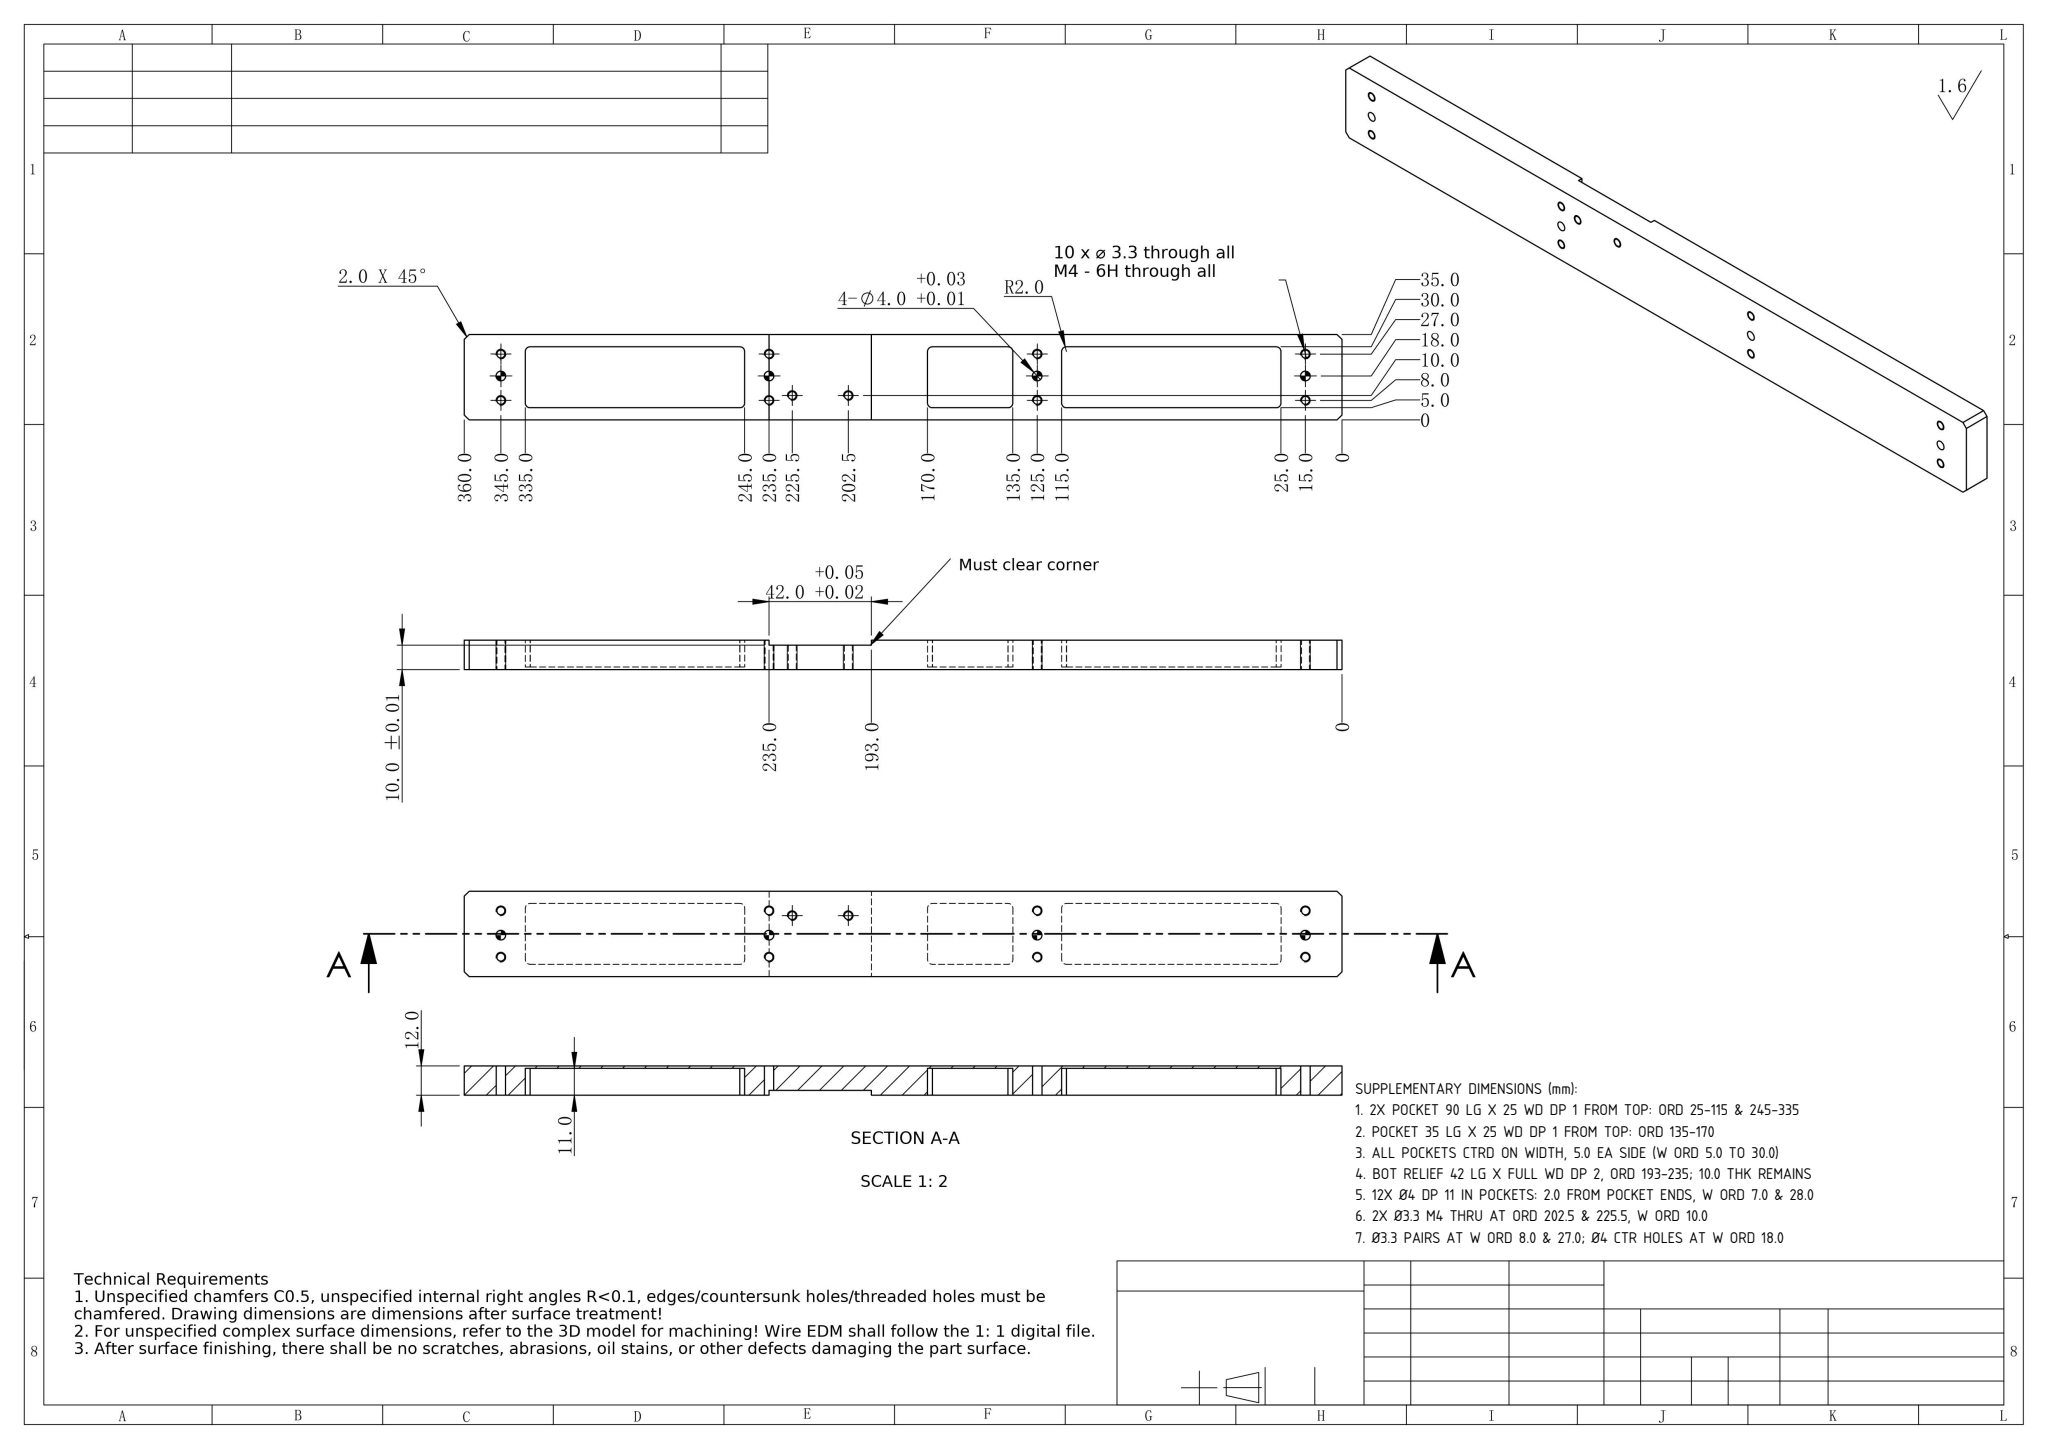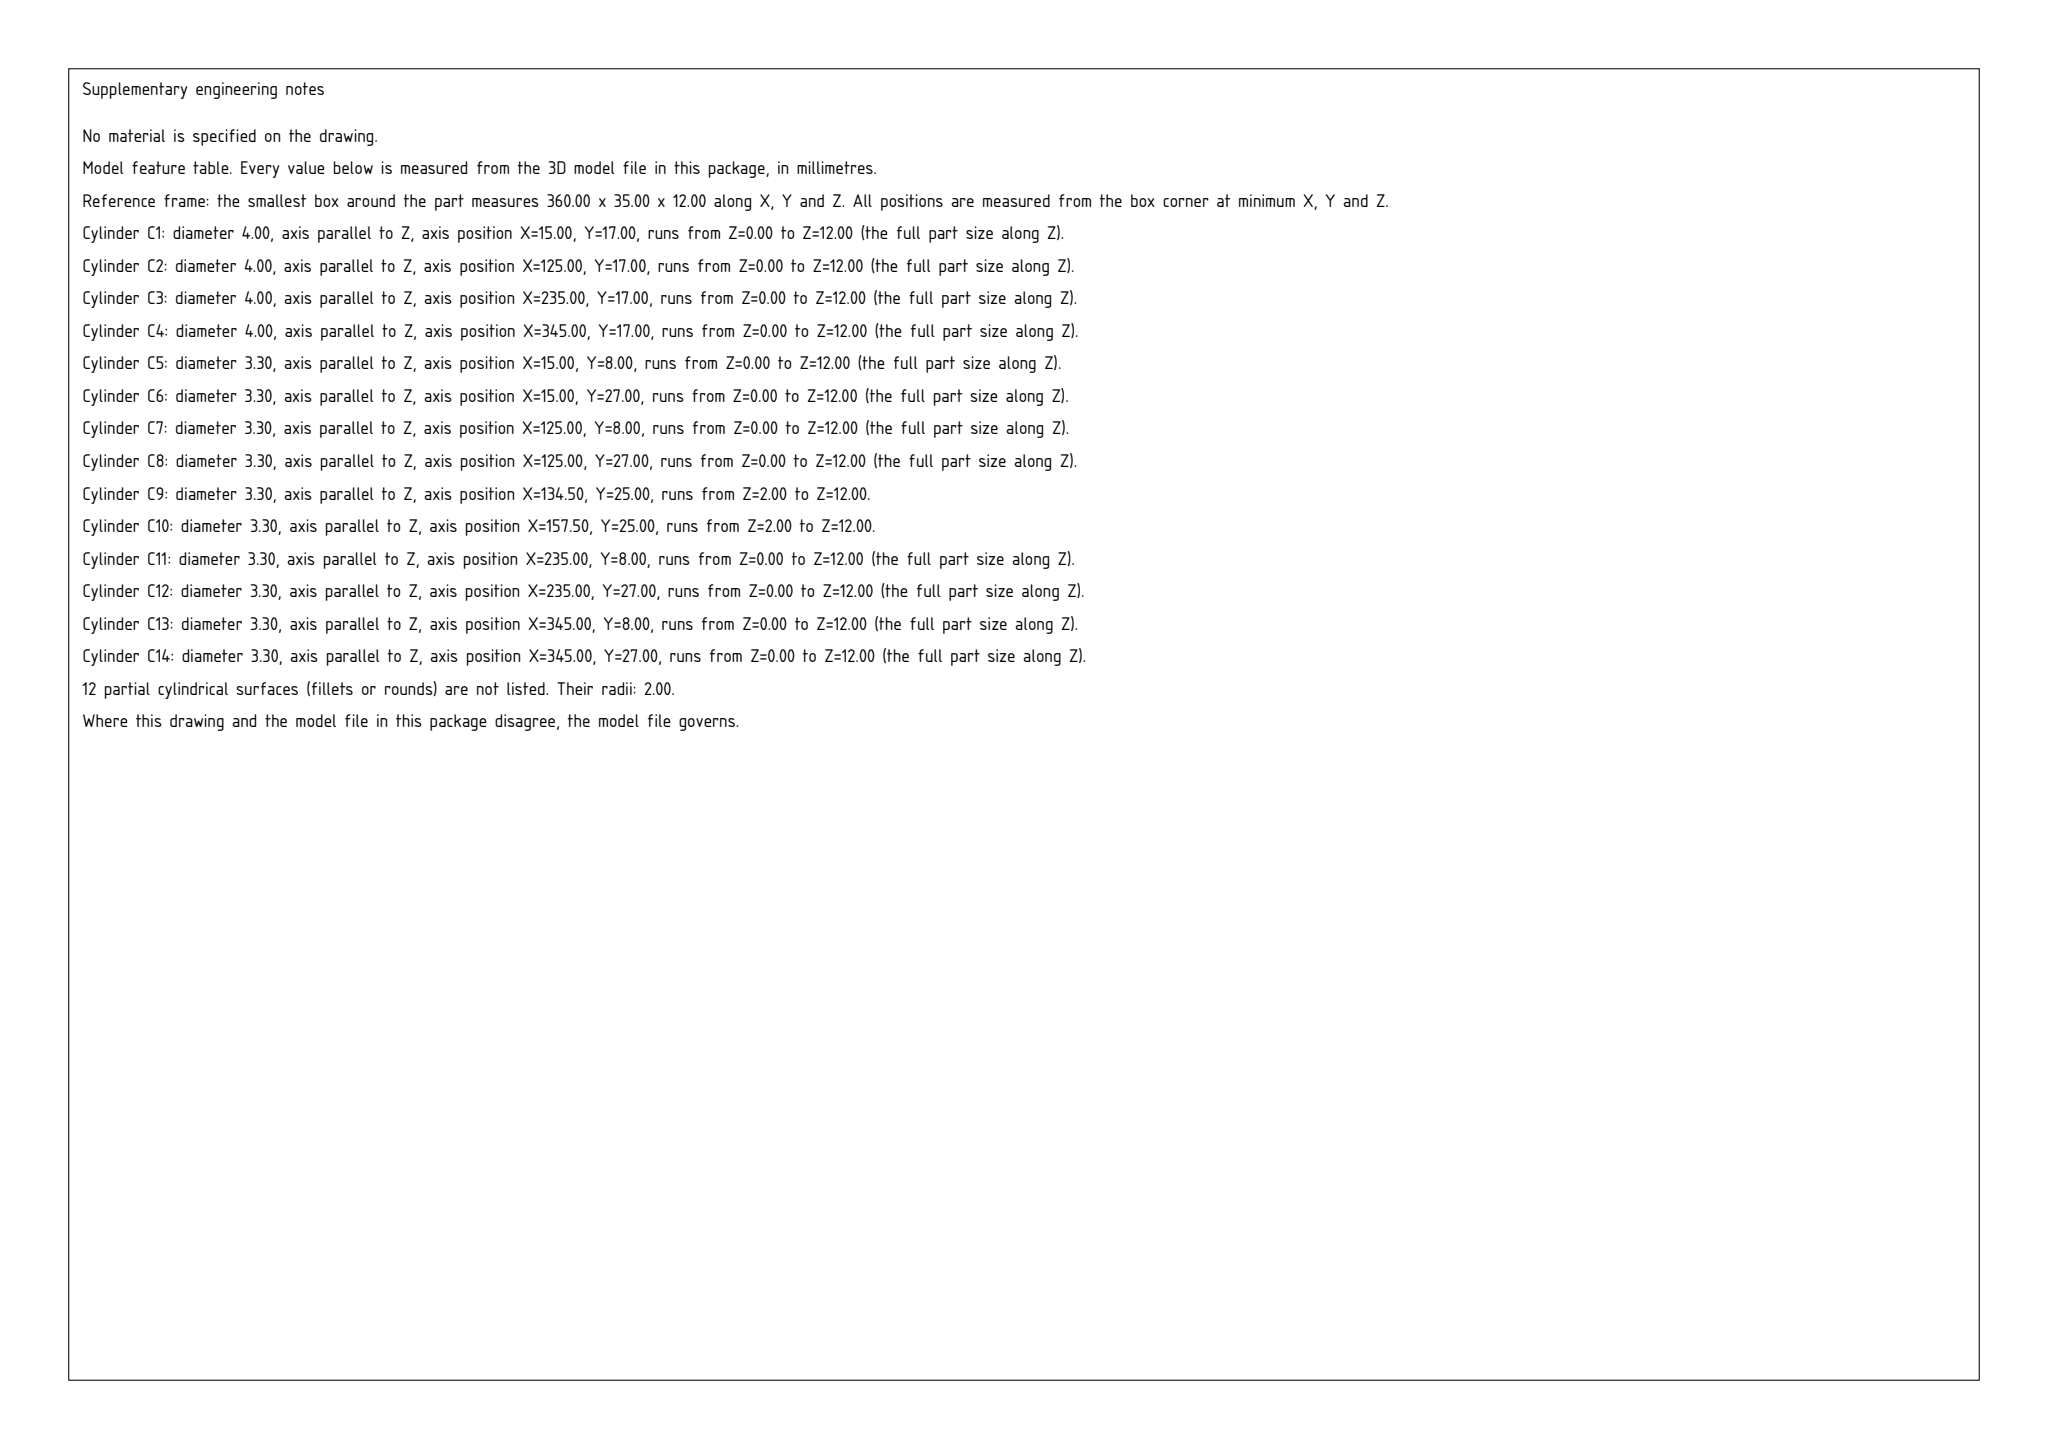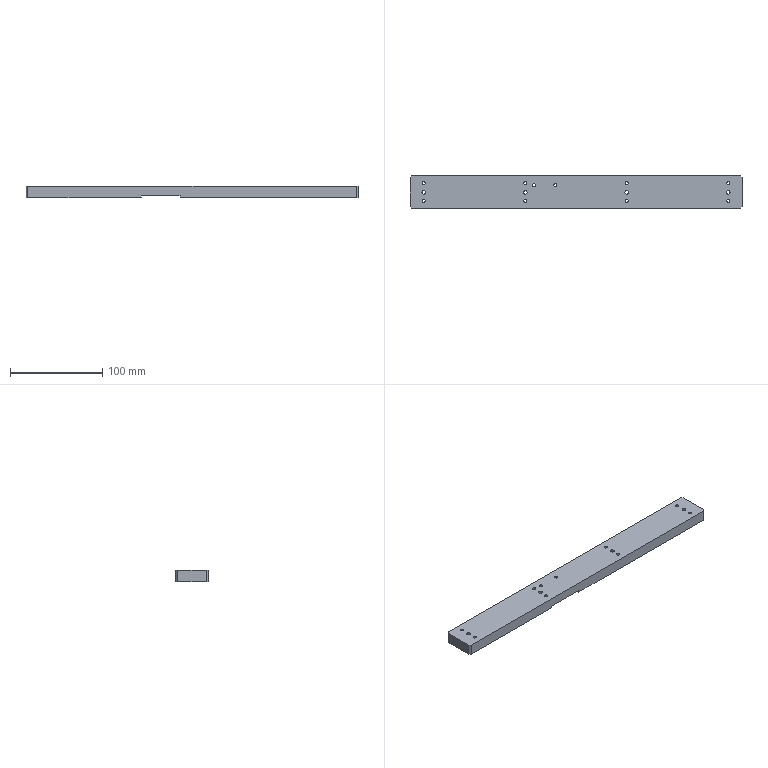Part | SolidWorks | mm | 1 solid | 72 faces | box 360 x 35 x 12 mm | volume 87587 mm3 | cylinder 40 | plane 32 | commonest cylinder face diameters 4 x20 3.3 x20
build123d program:
from build123d import *

# Parameters (mm, degrees)
SKETCH1_W           = 360
SKETCH1_H           = 35
BOSS_EXTRUDE1_DEPTH = 12
SKETCH2_W           = 42
SKETCH2_H           = 35
CUT_EXTRUDE1_DEPTH  = 2
M4_TAPPED_HOLE1_D   = 3.3
SKETCH6_W           = 90
SKETCH6_H           = 25
SKETCH6_W_2         = 35
CUT_EXTRUDE2_DEPTH  = 11
FILLET1_R           = 2
CHAMFER1_SIZE       = 2
SKETCH8_R           = 2
CUT_EXTRUDE3_DEPTH  = 362.896


with BuildPart() as part:
    # Sketch1 → Boss-Extrude1 (new body)
    with BuildSketch(Plane.XY):
        with Locations((180, 17.5)):
            Rectangle(SKETCH1_W, SKETCH1_H)
    extrude(amount=BOSS_EXTRUDE1_DEPTH)

    # Sketch2 → Cut-Extrude1 (cut)
    with BuildSketch(Plane(origin=(0, 0, 0), x_dir=(-1, 0, 0), z_dir=(0, 0, -1))):
        with Locations((-146, 17.5)):
            Rectangle(SKETCH2_W, SKETCH2_H)
    extrude(amount=-CUT_EXTRUDE1_DEPTH, mode=Mode.SUBTRACT)

    # M4 Tapped Hole1 (through all)
    with Locations(Plane(origin=(0, 0, 12), x_dir=(-1, 0, 0), z_dir=(0, 0, 1))):
        with Locations((-157.5, -25), (-134.5, -25), (-15, -27), (-15, -8), (-125, -27), (-125, -8), (-235, -27), (-235, -8), (-345, -27), (-345, -8)):
            Hole(M4_TAPPED_HOLE1_D / 2)

    # Sketch6 → Cut-Extrude2 (cut)
    with BuildSketch(Plane(origin=(0, 0, 0), x_dir=(-1, 0, 0), z_dir=(0, 0, -1))):
        with Locations((-290, 17.5)):
            Rectangle(SKETCH6_W, SKETCH6_H)
        with Locations((-70, 17.5)):
            Rectangle(SKETCH6_W, SKETCH6_H)
        with Locations((-207.5, 17.5)):
            Rectangle(SKETCH6_W_2, SKETCH6_H)
    extrude(amount=-CUT_EXTRUDE2_DEPTH, mode=Mode.SUBTRACT)

    # Fillet1
    fillet1_edges = [part.edges().sort_by_distance(p)[0] for p in [
        (335, 5, 5.5),
        (335, 30, 5.5),
        (245, 30, 5.5),
        (245, 5, 5.5),
        (115, 5, 5.5),
        (115, 30, 5.5),
        (25, 30, 5.5),
        (25, 5, 5.5),
        (225, 5, 5.5),
        (225, 30, 5.5),
        (190, 30, 5.5),
        (190, 5, 5.5),
    ]]
    fillet(fillet1_edges, radius=FILLET1_R)

    # Chamfer1
    chamfer1_edges = [part.edges().sort_by_distance(p)[0] for p in [
        (0, 35, 6),
        (360, 35, 6),
        (360, 0, 6),
        (0, 0, 6),
    ]]
    chamfer(chamfer1_edges, length=CHAMFER1_SIZE)

    # Sketch8 → Cut-Extrude3 (cut, through all)
    with BuildSketch(Plane.XY.offset(12)):
        with Locations((15, 17)):
            Circle(SKETCH8_R)
        with Locations((125, 17)):
            Circle(SKETCH8_R)
        with Locations((235, 17)):
            Circle(SKETCH8_R)
        with Locations((345, 17)):
            Circle(SKETCH8_R)
    extrude(amount=-CUT_EXTRUDE3_DEPTH, mode=Mode.SUBTRACT)


solid = part.part